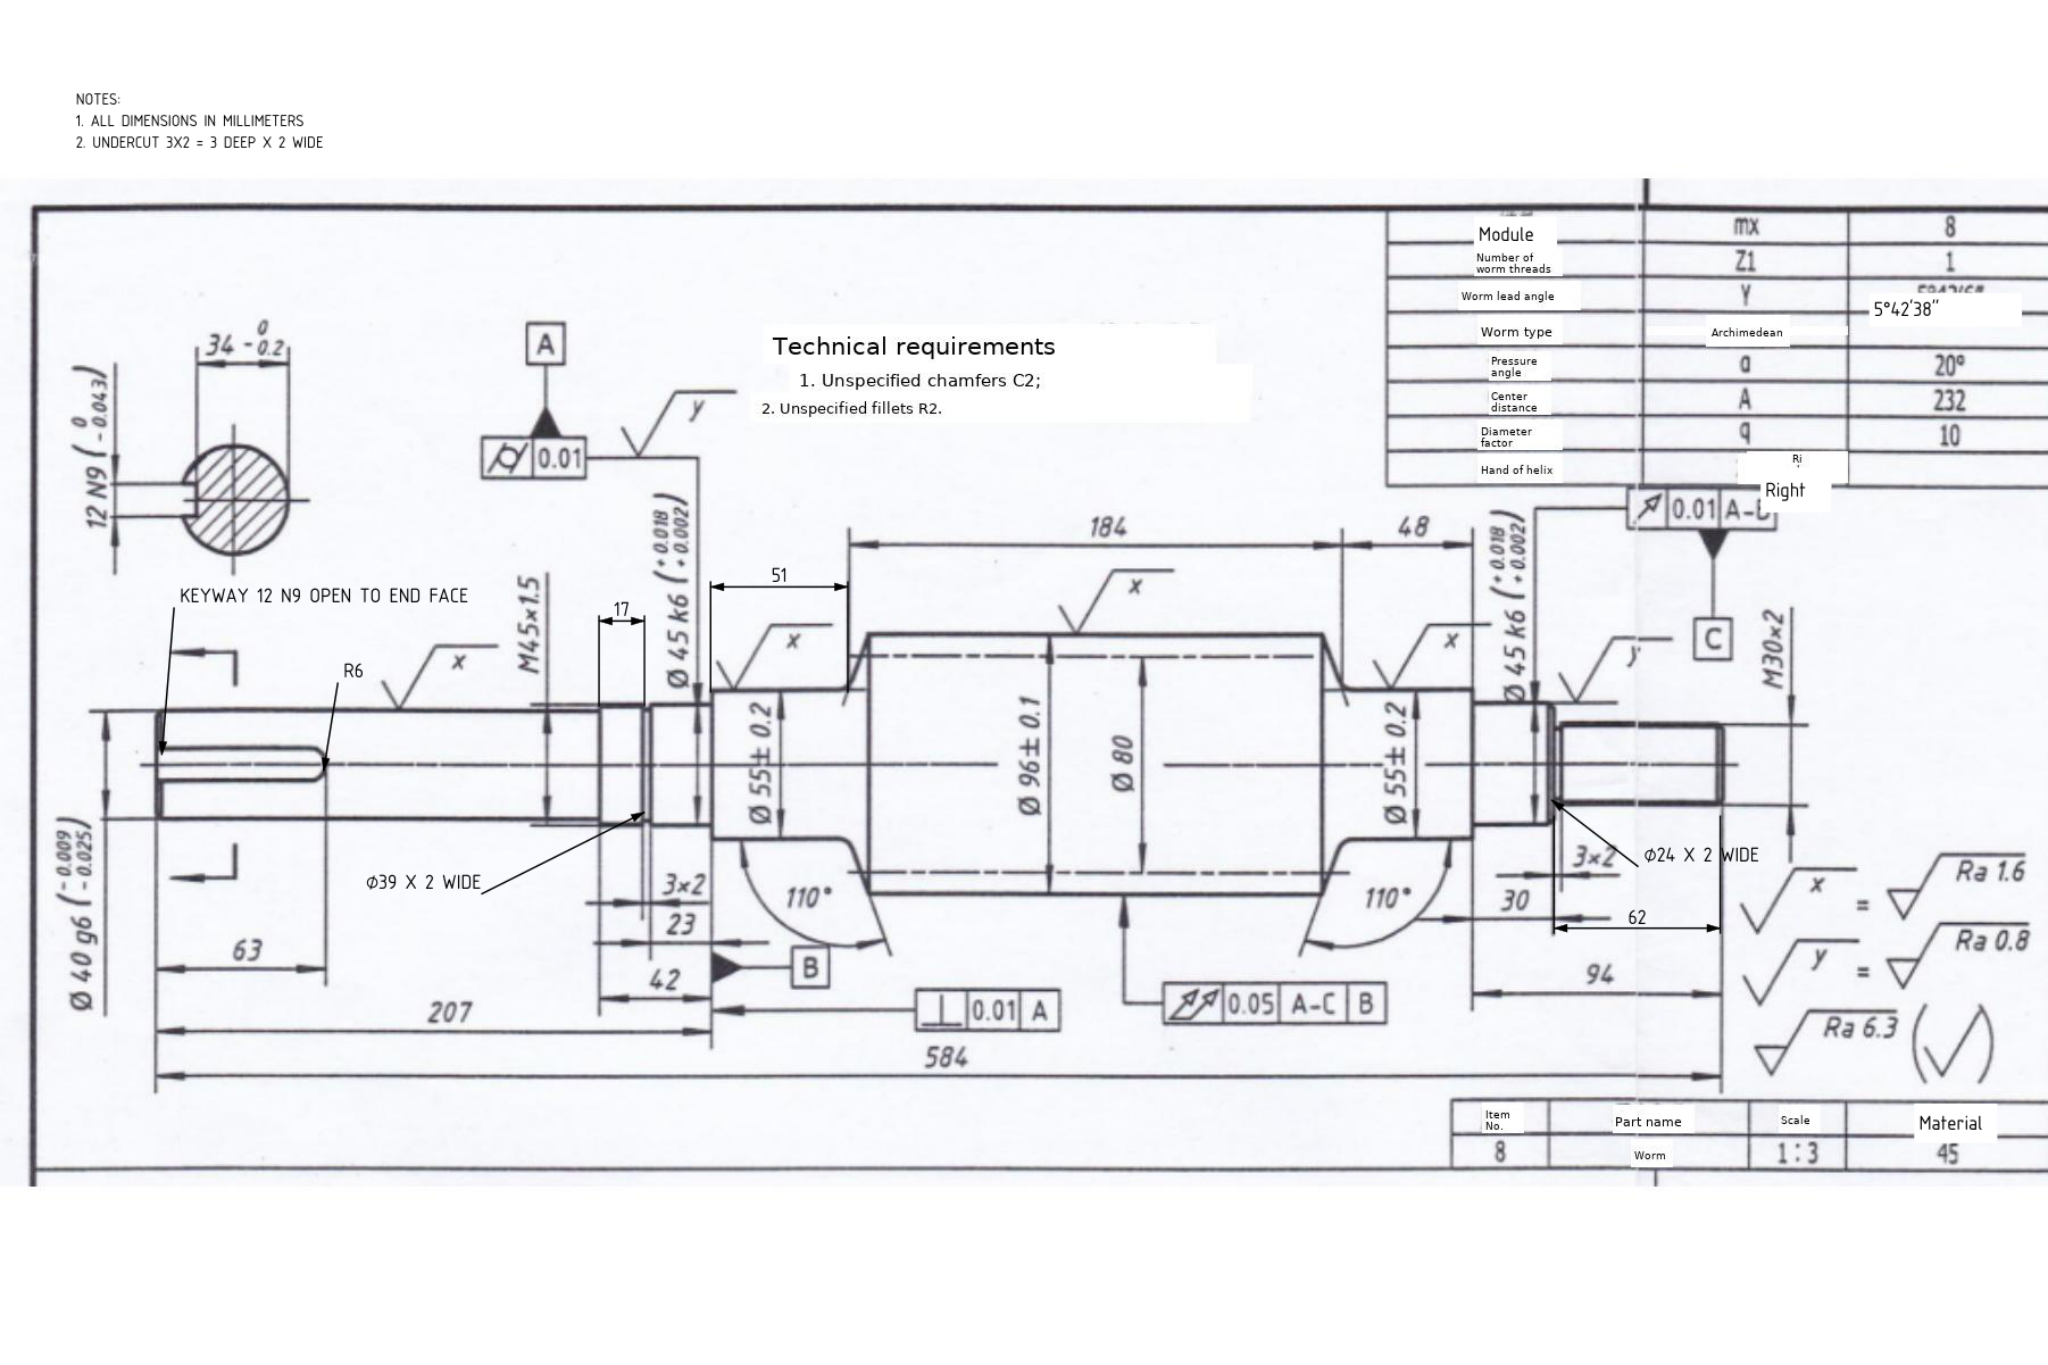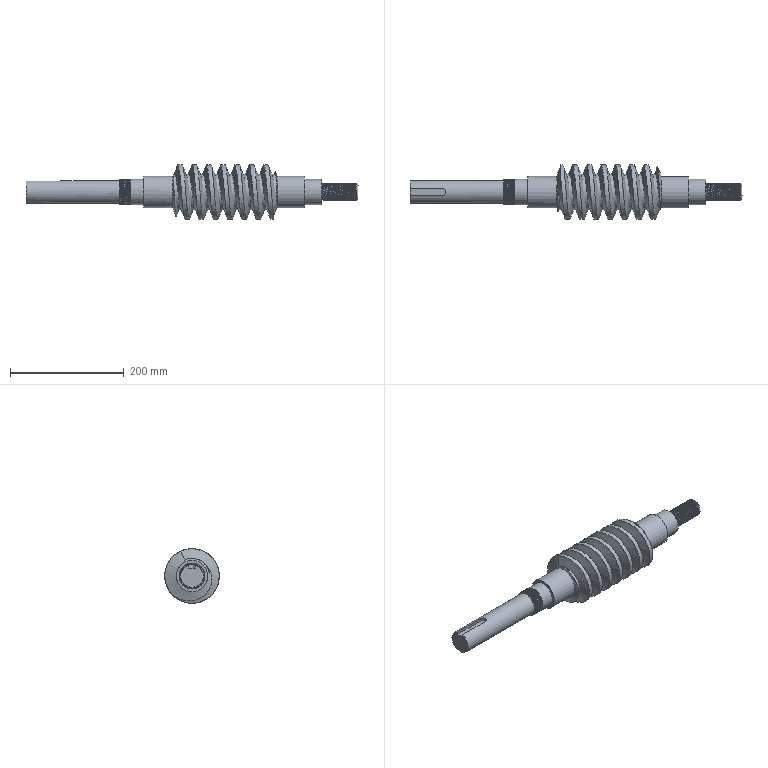Part | NX | mm | 1 solid | 36 faces | box 584 x 96.01 x 96.01 mm | volume 1537652 mm3 | plane 14 | cylinder 13 | spline 6 | cone 3 | commonest cylinder face diameters 45 x3 55 x2 40 x1 39 x1 96 x1 24 x1 30 x1 43.5 x1